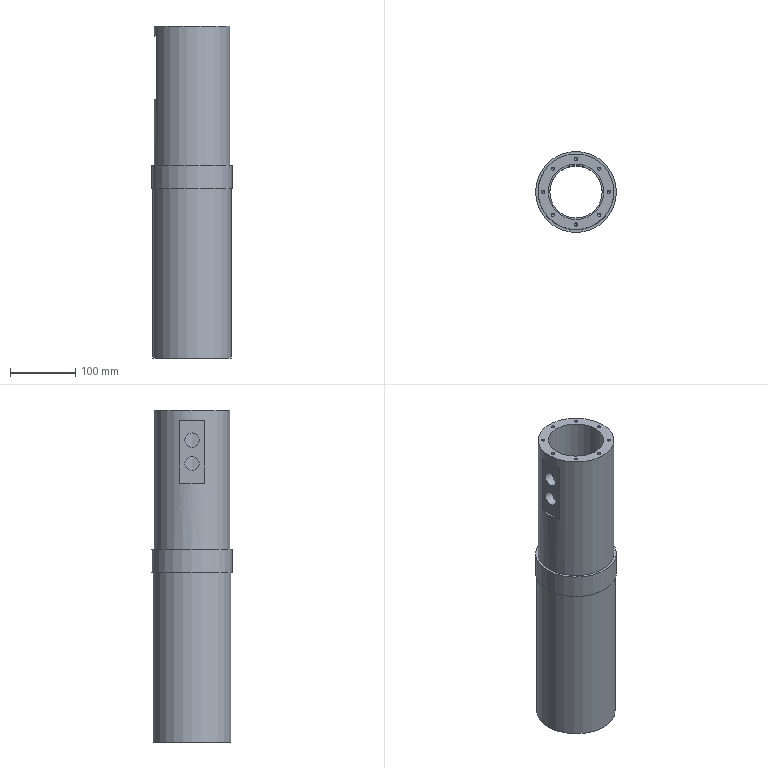Component | NX | CH3404_8_2-1 | 1 solid | 39 faces | volume 2753495 mm3 | cylinder 19 | plane 12 | cone 8 | commonest cylinder face diameters 5 x8 22 x2 116 x1 124 x1 120 x1 101 x1 95 x1 80 x1